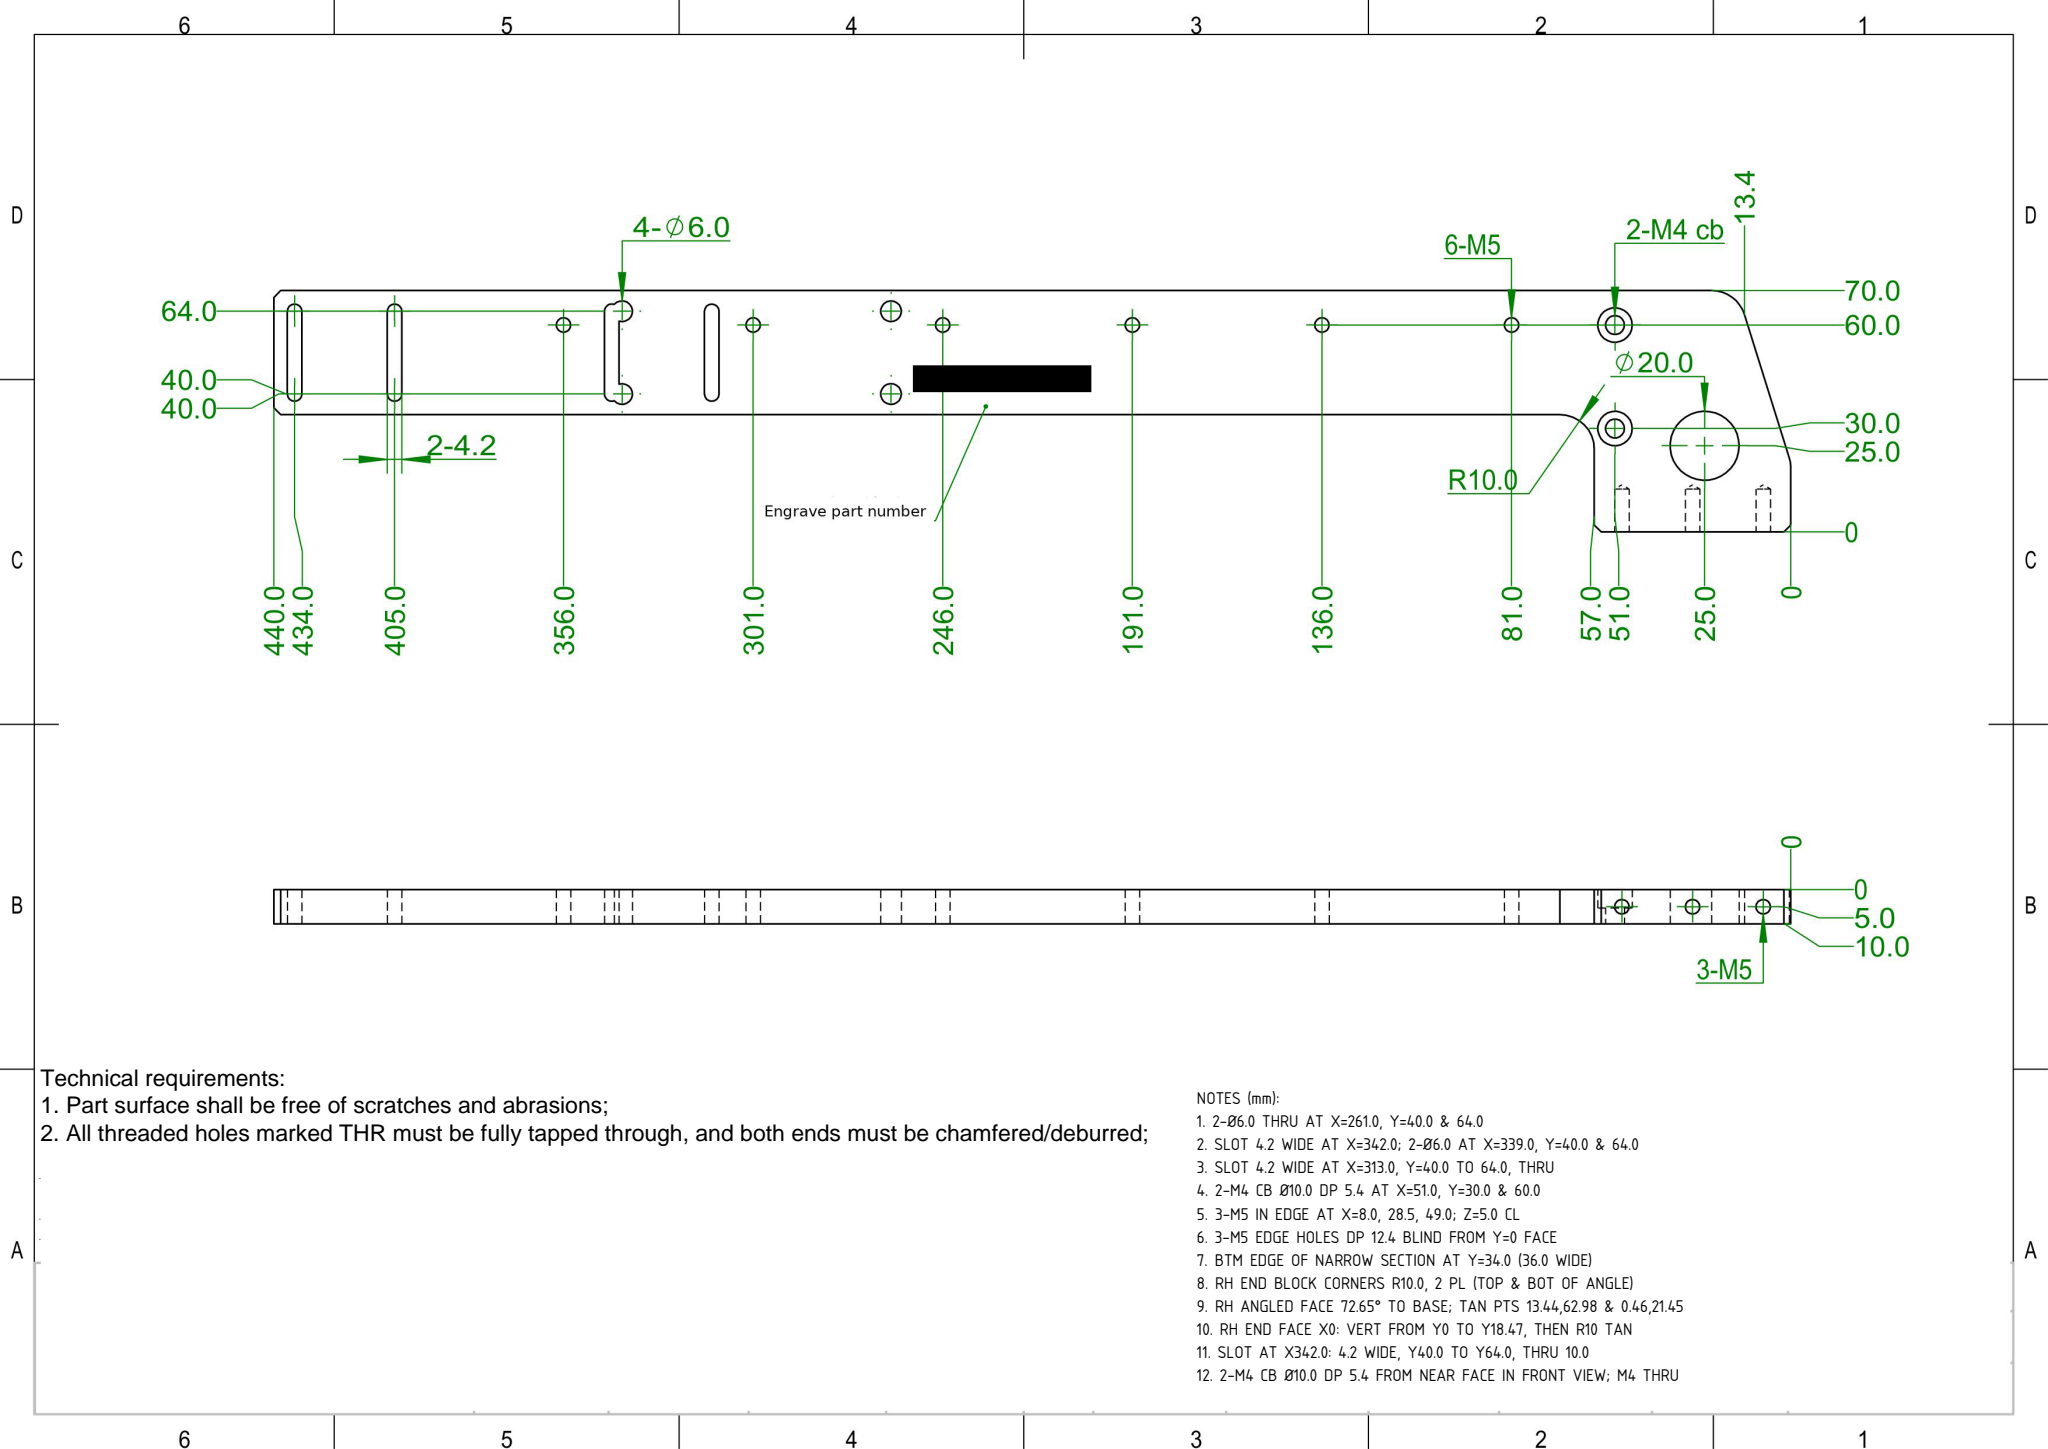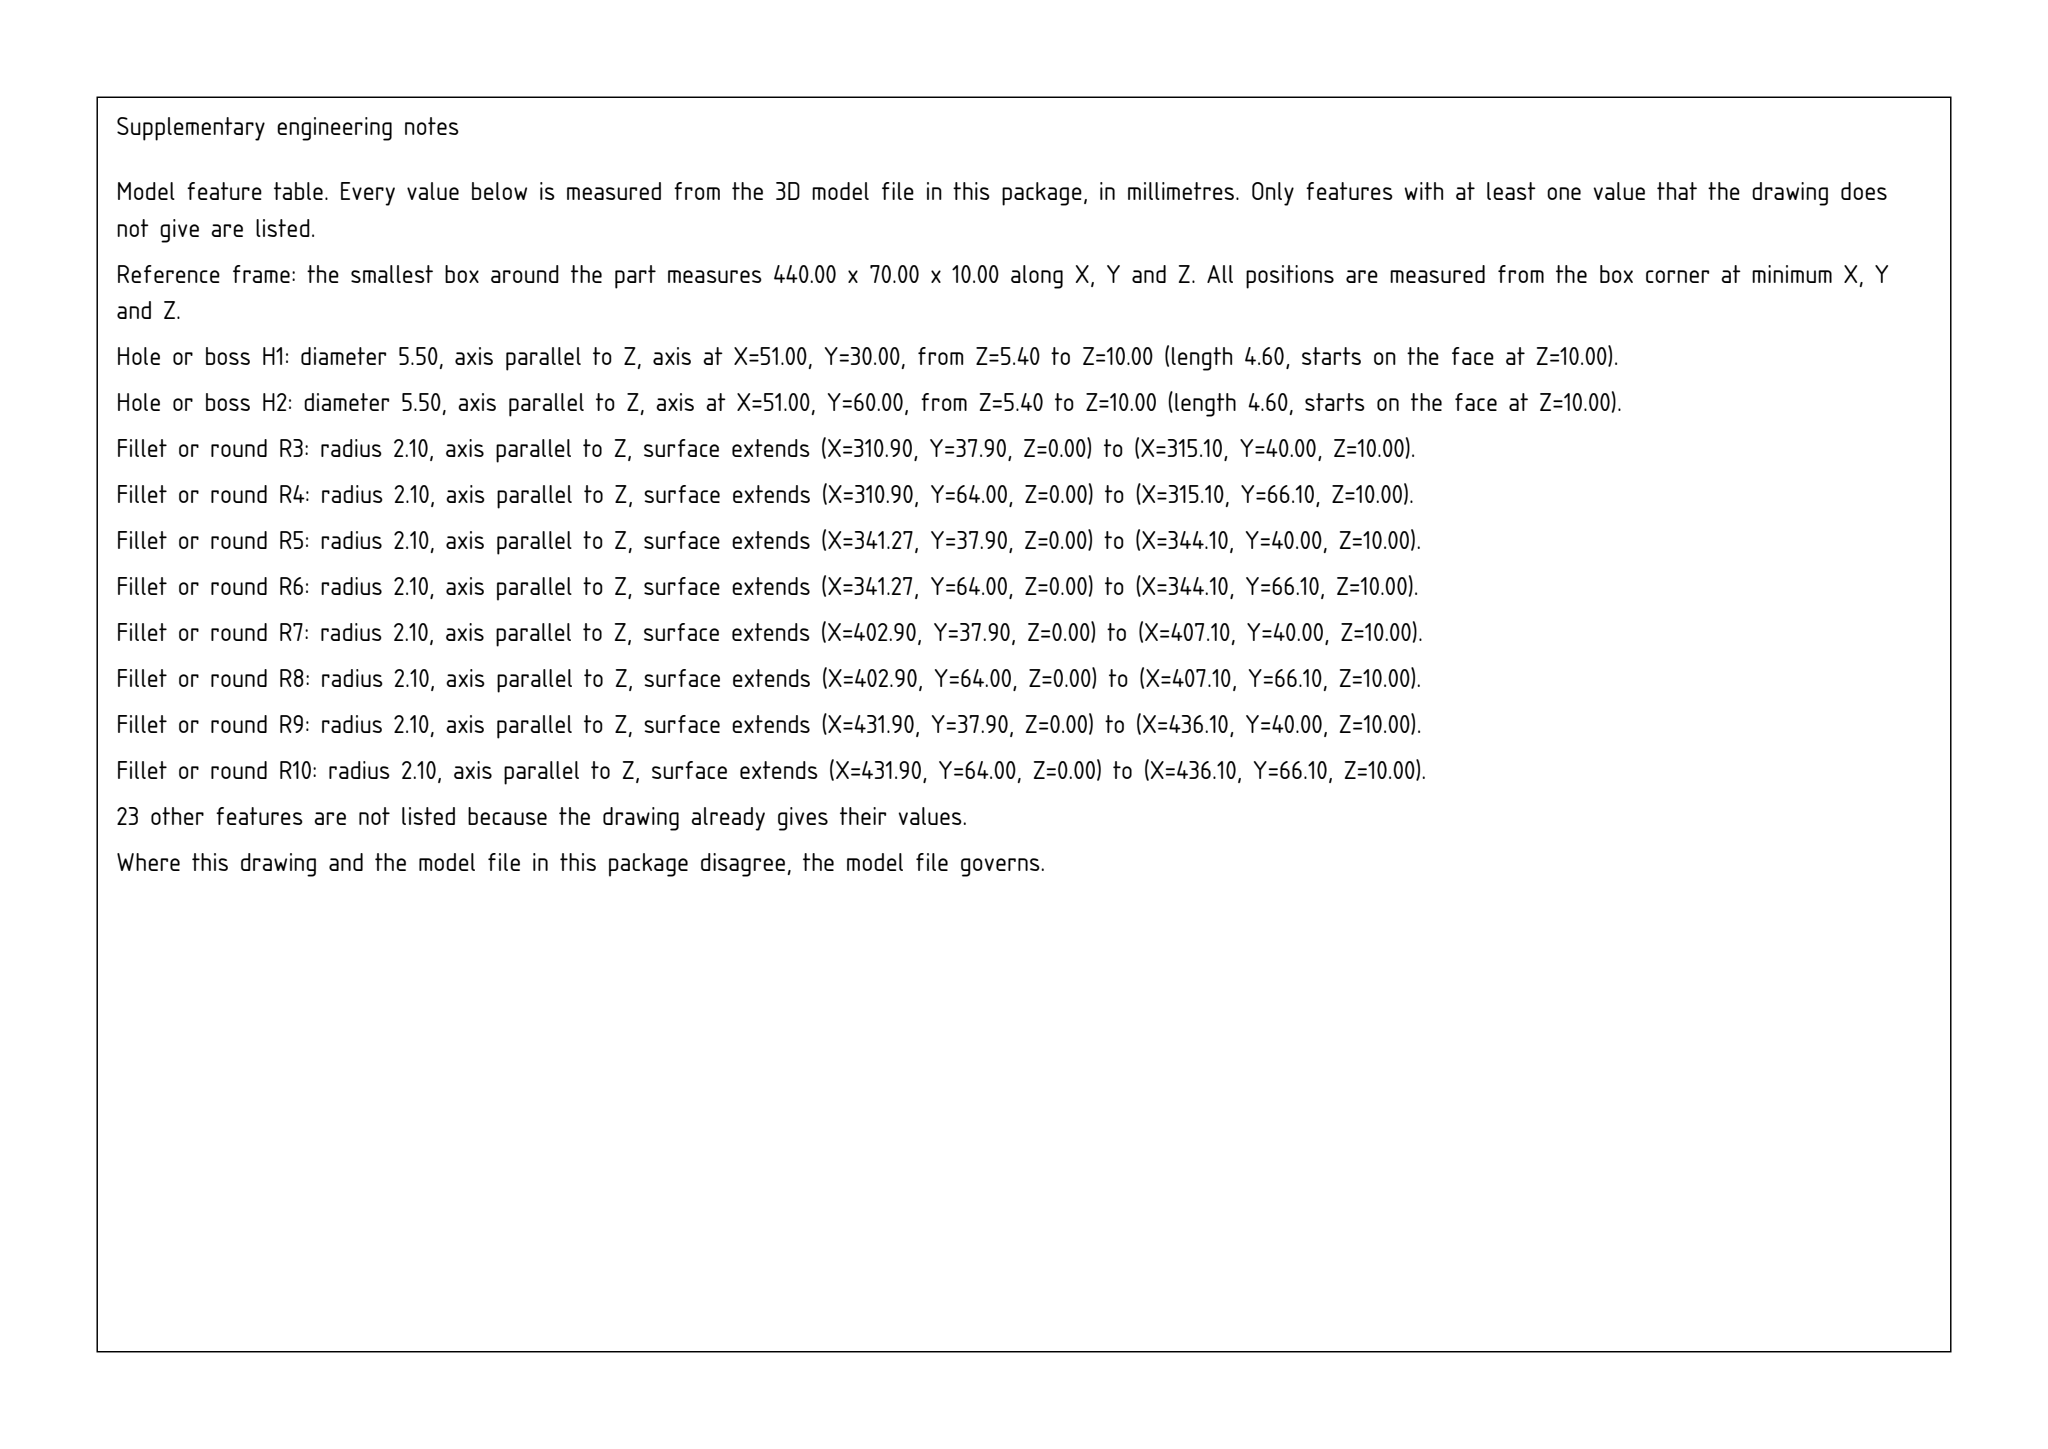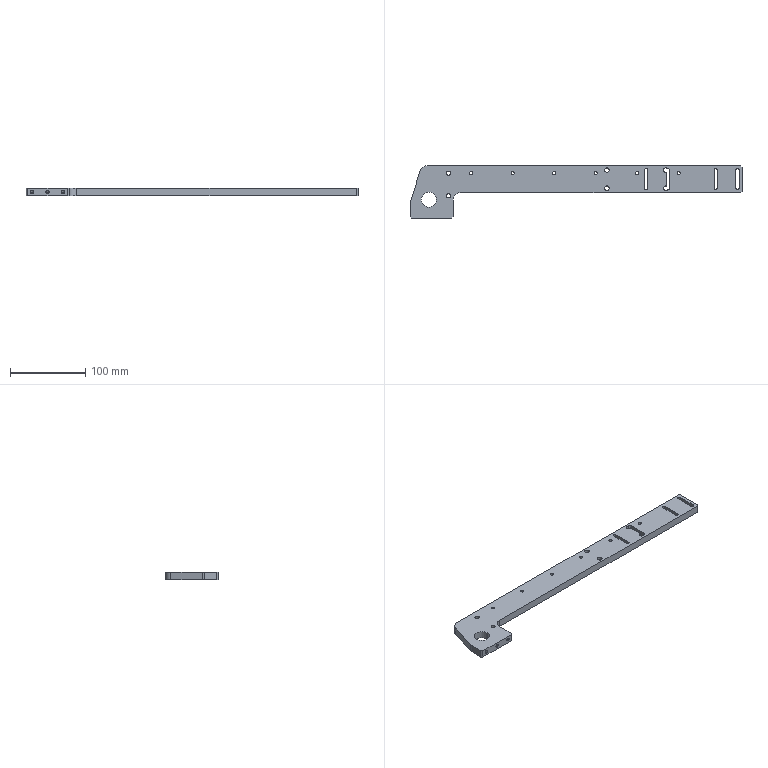Part | SolidWorks | mm | 1 solid | 74 faces | box 440 x 70 x 10 mm | volume 162764 mm3 | cylinder 45 | plane 23 | cone 6 | commonest cylinder face diameters 4.2 x26 6 x6 20 x5 5.5 x4 10 x4
Drawing notes:
2-Ø6.0 THRU AT X=261.0, Y=40.0 & 64.0 | from the solid: cyl dia 6.0 axis z at [261.0,40.0] and [261.0,64.0], len 10.0
SLOT 4.2 WIDE AT X=342.0; 2-Ø6.0 AT X=339.0, Y=40.0 & 64.0 | from the solid: x-planes 339.9/344.1 (4.2 wide) with Ø4.2 at [342,40]&[342,64]; Ø6.0 at [339,40]&[339,64]
SLOT 4.2 WIDE AT X=313.0, Y=40.0 TO 64.0, THRU | from the solid: x-planes 310.9/315.1 (4.2 wide); Ø4.2 holes at [313,40] and [313,64], len 10.0
2-M4 CB Ø10.0 DP 5.4 AT X=51.0, Y=30.0 & 60.0 | from the solid: cyl dia 10.0 axis z at [51,30] & [51,60] len 5.4 over dia 5.5 len 4.6; z-plane 5.4
3-M5 IN EDGE AT X=8.0, 28.5, 49.0; Z=5.0 CL | from the solid: cyl dia 4.2 axis y at [8,-,5], [28.5,-,5], [49,-,5]
3-M5 EDGE HOLES DP 12.4 BLIND FROM Y=0 FACE | from the solid: cyl dia 4.2 axis y length 12.4, y-plane 0.0
BTM EDGE OF NARROW SECTION AT Y=34.0 (36.0 WIDE) | from the solid: y-planes 0.0, 34.0, 70.0
RH END BLOCK CORNERS R10.0, 2 PL (TOP & BOT OF ANGLE) | from the solid: dia 20.0 axis z round at [22.98,60.0] and [10.0,18.47], len 10.0
RH ANGLED FACE 72.65° TO BASE; TAN PTS 13.44,62.98 & 0.46,21.45 | from the solid: Common ext tangent to R10 cyls at (10,18.47) & (22.98,60): dir (12.98,41.53) = 72.65 deg to X; tan pts (0.46,21.45) & (13.44,62.98)
RH END FACE X0: VERT FROM Y0 TO Y18.47, THEN R10 TAN | from the solid: Plane x=0.0 with R10 cyl centre (10.0,18.47) tangent to it at y=18.47; plane y=0.0 lower edge
SLOT AT X342.0: 4.2 WIDE, Y40.0 TO Y64.0, THRU 10.0 | from the solid: Planes x=339.9 & x=344.1 (4.2 wide); Ø4.2 z-cyls at (342,40) & (342,64), len 10.0 = full thk
2-M4 CB Ø10.0 DP 5.4 FROM NEAR FACE IN FRONT VIEW; M4 THRU | from the solid: Ø10 z-cyls at (51,30) & (51,60) len 5.4 ending on plane z=5.4 from z=10.0 face; Ø5.5 len 4.6 to z=0